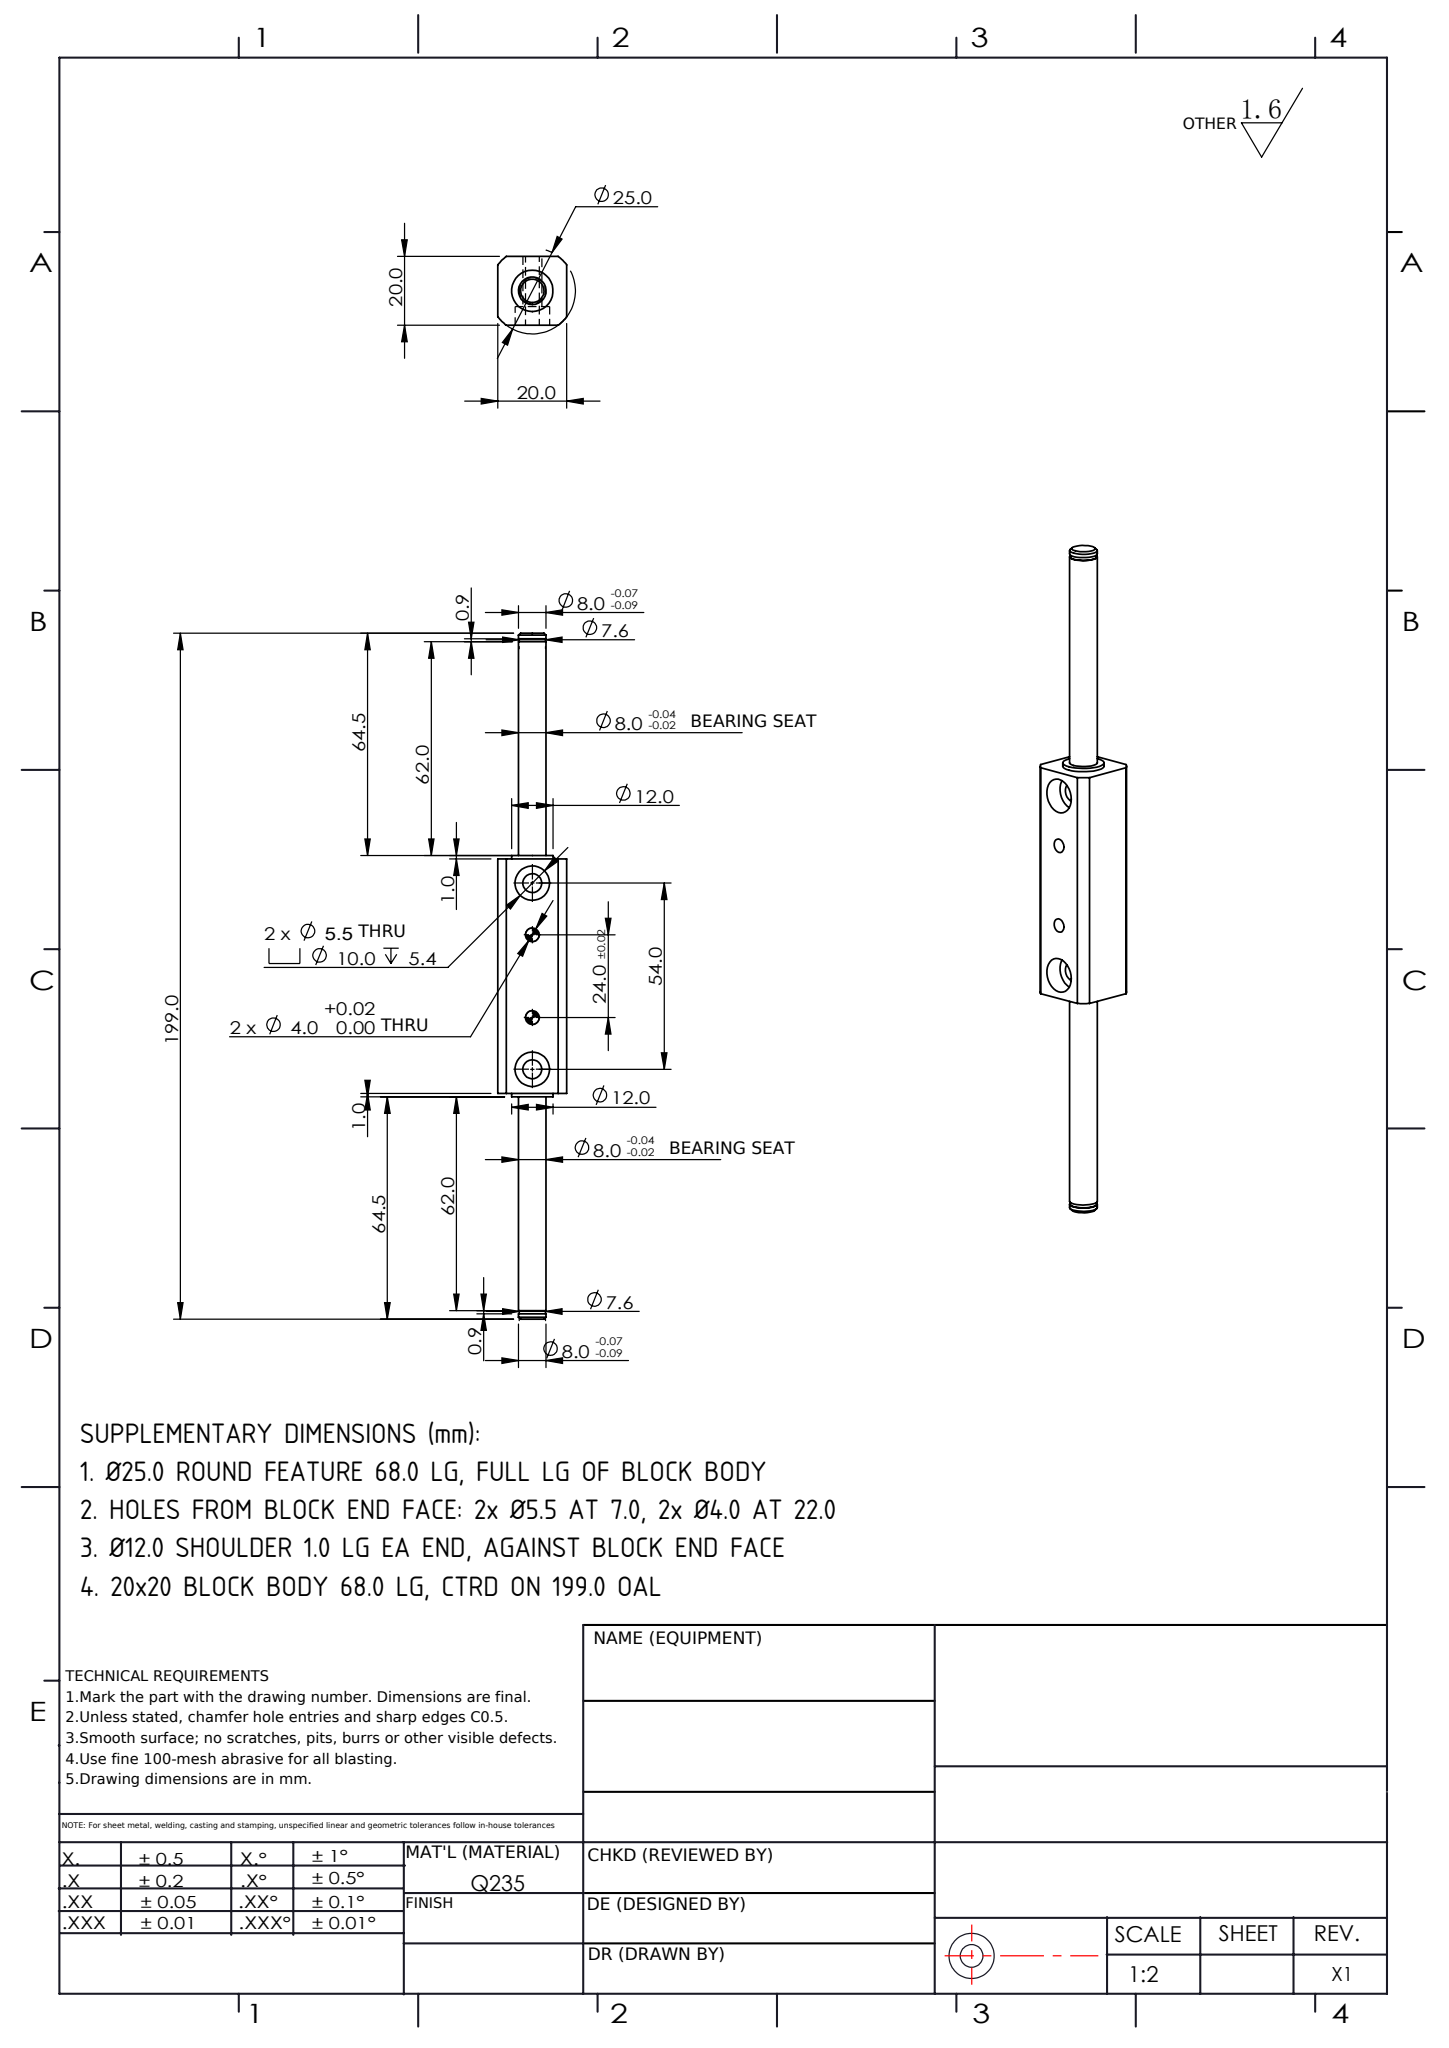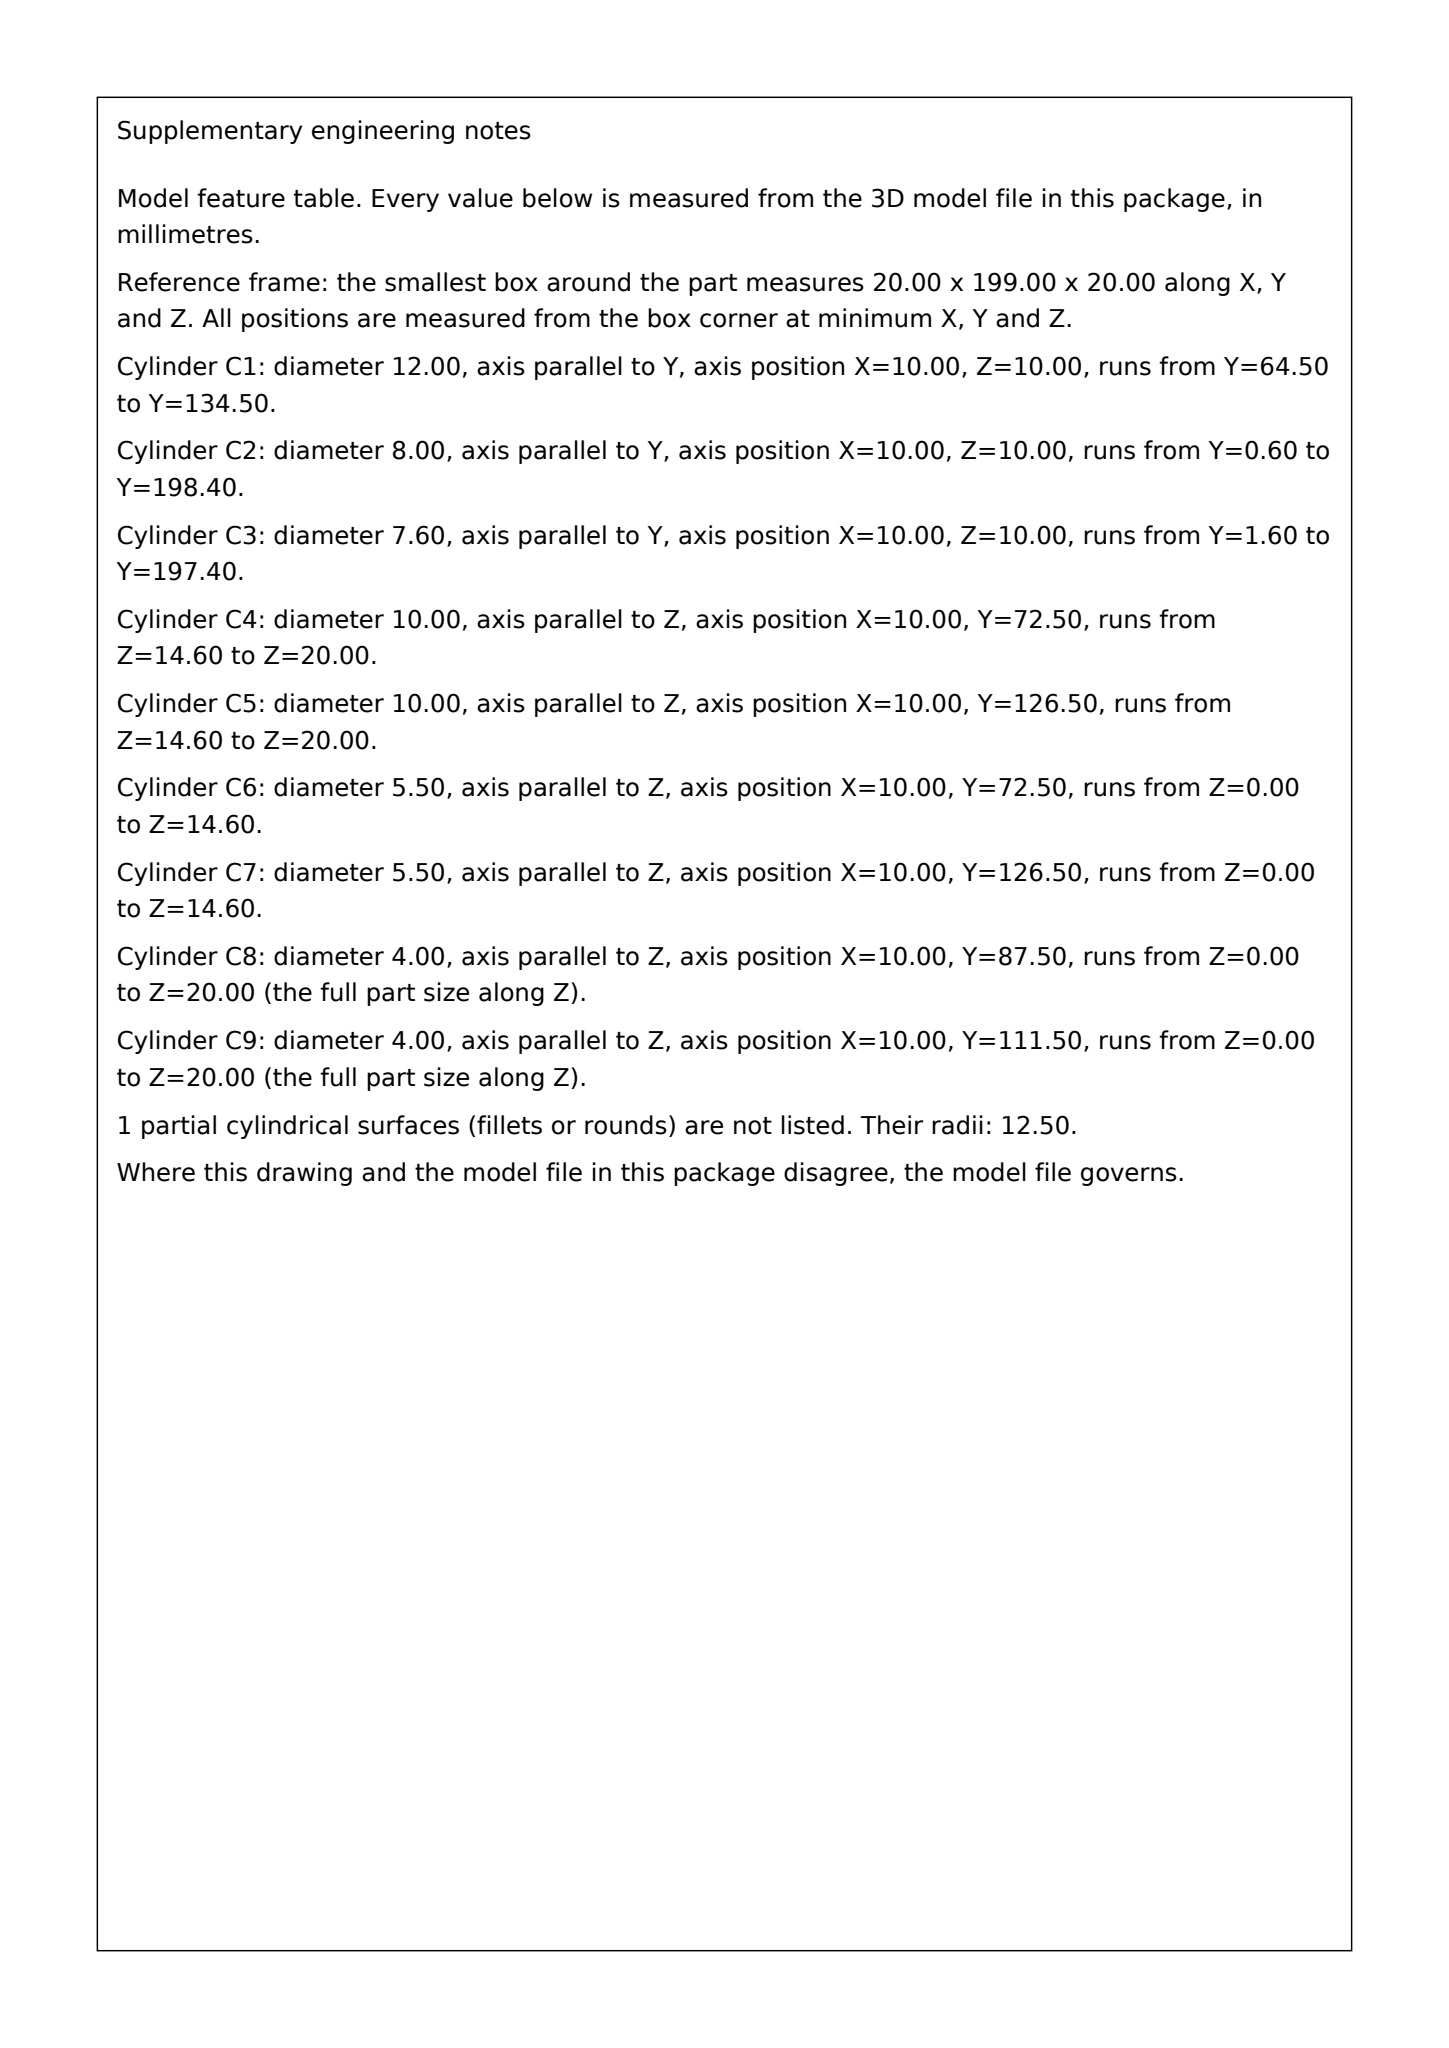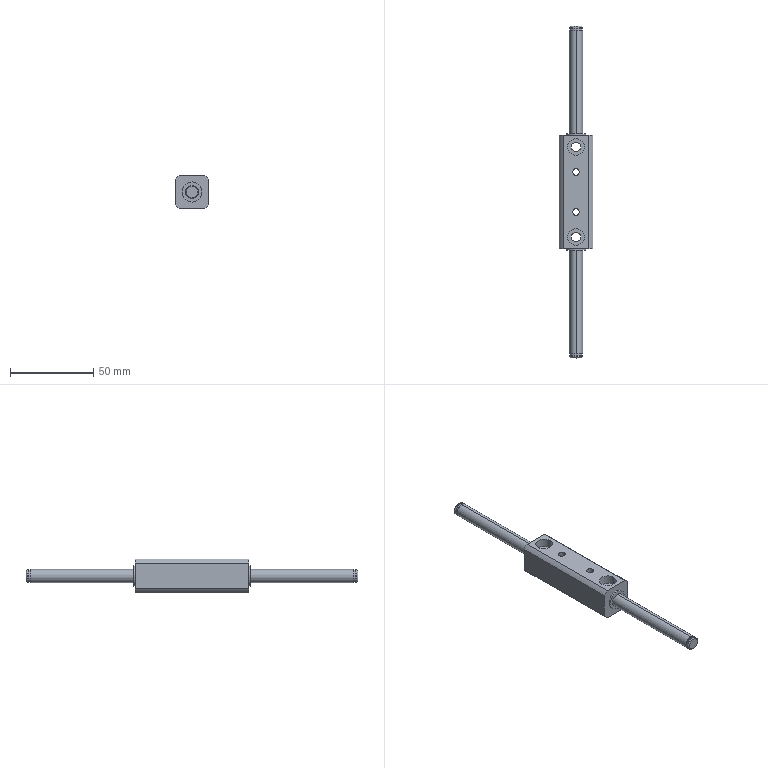Part | SolidWorks | mm | 1 solid | 52 faces | box 20 x 199 x 20 mm | volume 31079 mm3 | cylinder 32 | plane 16 | cone 4 | commonest cylinder face diameters 8 x8 7.6 x4 4 x4 10 x4 5.5 x4 12 x4 25 x4
build123d program:
from build123d import *

# Parameters (mm, degrees)
SKETCH1_W                                       = 20
SKETCH1_H                                       = 20
BOSS_EXTRUDE1_DEPTH                             = 68
SKETCH2_OUTSIDE_W                               = 36.73
SKETCH2_OUTSIDE_H                               = 36.73
SKETCH2_OUTSIDE_R                               = 12.5
CUT_EXTRUDE1_DEPTH                              = 70.455
SKETCH3_R                                       = 6
BOSS_EXTRUDE2_DEPTH                             = 1
SKETCH4_R                                       = 4
BOSS_EXTRUDE3_DEPTH                             = 64.5
BOSS_EXTRUDE4_START                             = 1
SKETCH5_R                                       = 6
BOSS_EXTRUDE4_DEPTH                             = 1
BOSS_EXTRUDE5_START                             = 64.5
SKETCH6_R                                       = 4
BOSS_EXTRUDE5_DEPTH                             = 64.5
M5_HEX_SOCKET_HEAD_CAP_SCREW_CBORE1_D           = 5.5
M5_HEX_SOCKET_HEAD_CAP_SCREW_CBORE1_CBORE_D     = 10
M5_HEX_SOCKET_HEAD_CAP_SCREW_CBORE1_CBORE_DEPTH = 5.4
HOLE1_D                                         = 4
SKETCH11_W                                      = 0.2
SKETCH11_H                                      = 0.9
CHAMFER1_SIZE                                   = 0.6


with BuildPart() as part:
    # Sketch1 → Boss-Extrude1 (new body)
    with BuildSketch(Plane(origin=(0, 0, 0), x_dir=(1, 0, 0), z_dir=(0, 1, 0))):
        Rectangle(SKETCH1_W, SKETCH1_H)
    extrude(amount=BOSS_EXTRUDE1_DEPTH)

    # Sketch2 outside → Cut-Extrude1 (cut, through all)
    with BuildSketch(Plane(origin=(0, 68, 0), x_dir=(1, 0, 0), z_dir=(0, 1, 0))):
        Rectangle(SKETCH2_OUTSIDE_W, SKETCH2_OUTSIDE_H)
        Circle(SKETCH2_OUTSIDE_R, mode=Mode.SUBTRACT)
    extrude(amount=-CUT_EXTRUDE1_DEPTH, mode=Mode.SUBTRACT)

    # Sketch3 → Boss-Extrude2 (add)
    with BuildSketch(Plane(origin=(0, 68, 0), x_dir=(1, 0, 0), z_dir=(0, 1, 0))):
        with Locations(Location((0, 0, 0), (0, 0, 270))):
            Circle(SKETCH3_R)
    extrude(amount=BOSS_EXTRUDE2_DEPTH)

    # Sketch4 → Boss-Extrude3 (add)
    with BuildSketch(Plane(origin=(0, 69, 0), x_dir=(1, 0, 0), z_dir=(0, 1, 0))):
        with Locations(Location((0, 0, 0), (0, 0, 270))):
            Circle(SKETCH4_R)
    extrude(amount=BOSS_EXTRUDE3_DEPTH)

    # Sketch5 → Boss-Extrude4 (add)
    with BuildSketch(Plane.XZ.offset(BOSS_EXTRUDE4_START)):
        with Locations(Location((0, 0, 0), (0, 0, 90))):
            Circle(SKETCH5_R)
    extrude(amount=-BOSS_EXTRUDE4_DEPTH)

    # Sketch6 → Boss-Extrude5 (add)
    with BuildSketch(Plane.XZ.offset(1).offset(BOSS_EXTRUDE5_START)):
        with Locations(Location((0, 0, 0), (0, 0, 90))):
            Circle(SKETCH6_R)
    extrude(amount=-BOSS_EXTRUDE5_DEPTH)

    # M5 Hex Socket Head Cap Screw CBORE1 (through all)
    with Locations(Plane.XY.offset(10)):
        with Locations((0, 61), (0, 7)):
            CounterBoreHole(M5_HEX_SOCKET_HEAD_CAP_SCREW_CBORE1_D / 2, M5_HEX_SOCKET_HEAD_CAP_SCREW_CBORE1_CBORE_D / 2, M5_HEX_SOCKET_HEAD_CAP_SCREW_CBORE1_CBORE_DEPTH)

    # Hole1 (through all)
    with Locations(Plane.XY.offset(10)):
        with Locations((0, 46), (0, 22)):
            Hole(HOLE1_D / 2)

    # Sketch11 → Cut-Revolve1 (revolve, cut)
    with BuildSketch(Plane.XY):
        with Locations((-3.9, 131.45)):
            Rectangle(SKETCH11_W, SKETCH11_H)
        with Locations((-3.9, -63.45)):
            Rectangle(SKETCH11_W, SKETCH11_H)
    revolve(axis=Axis((0, 133.5, 0), (0, -1, 0)), mode=Mode.SUBTRACT)

    # Chamfer1
    chamfer1_edges = [part.edges().sort_by_distance(p)[0] for p in [
        (0, 133.5, -4),
        (0, -65.5, -4),
    ]]
    chamfer(chamfer1_edges, length=CHAMFER1_SIZE)


solid = part.part